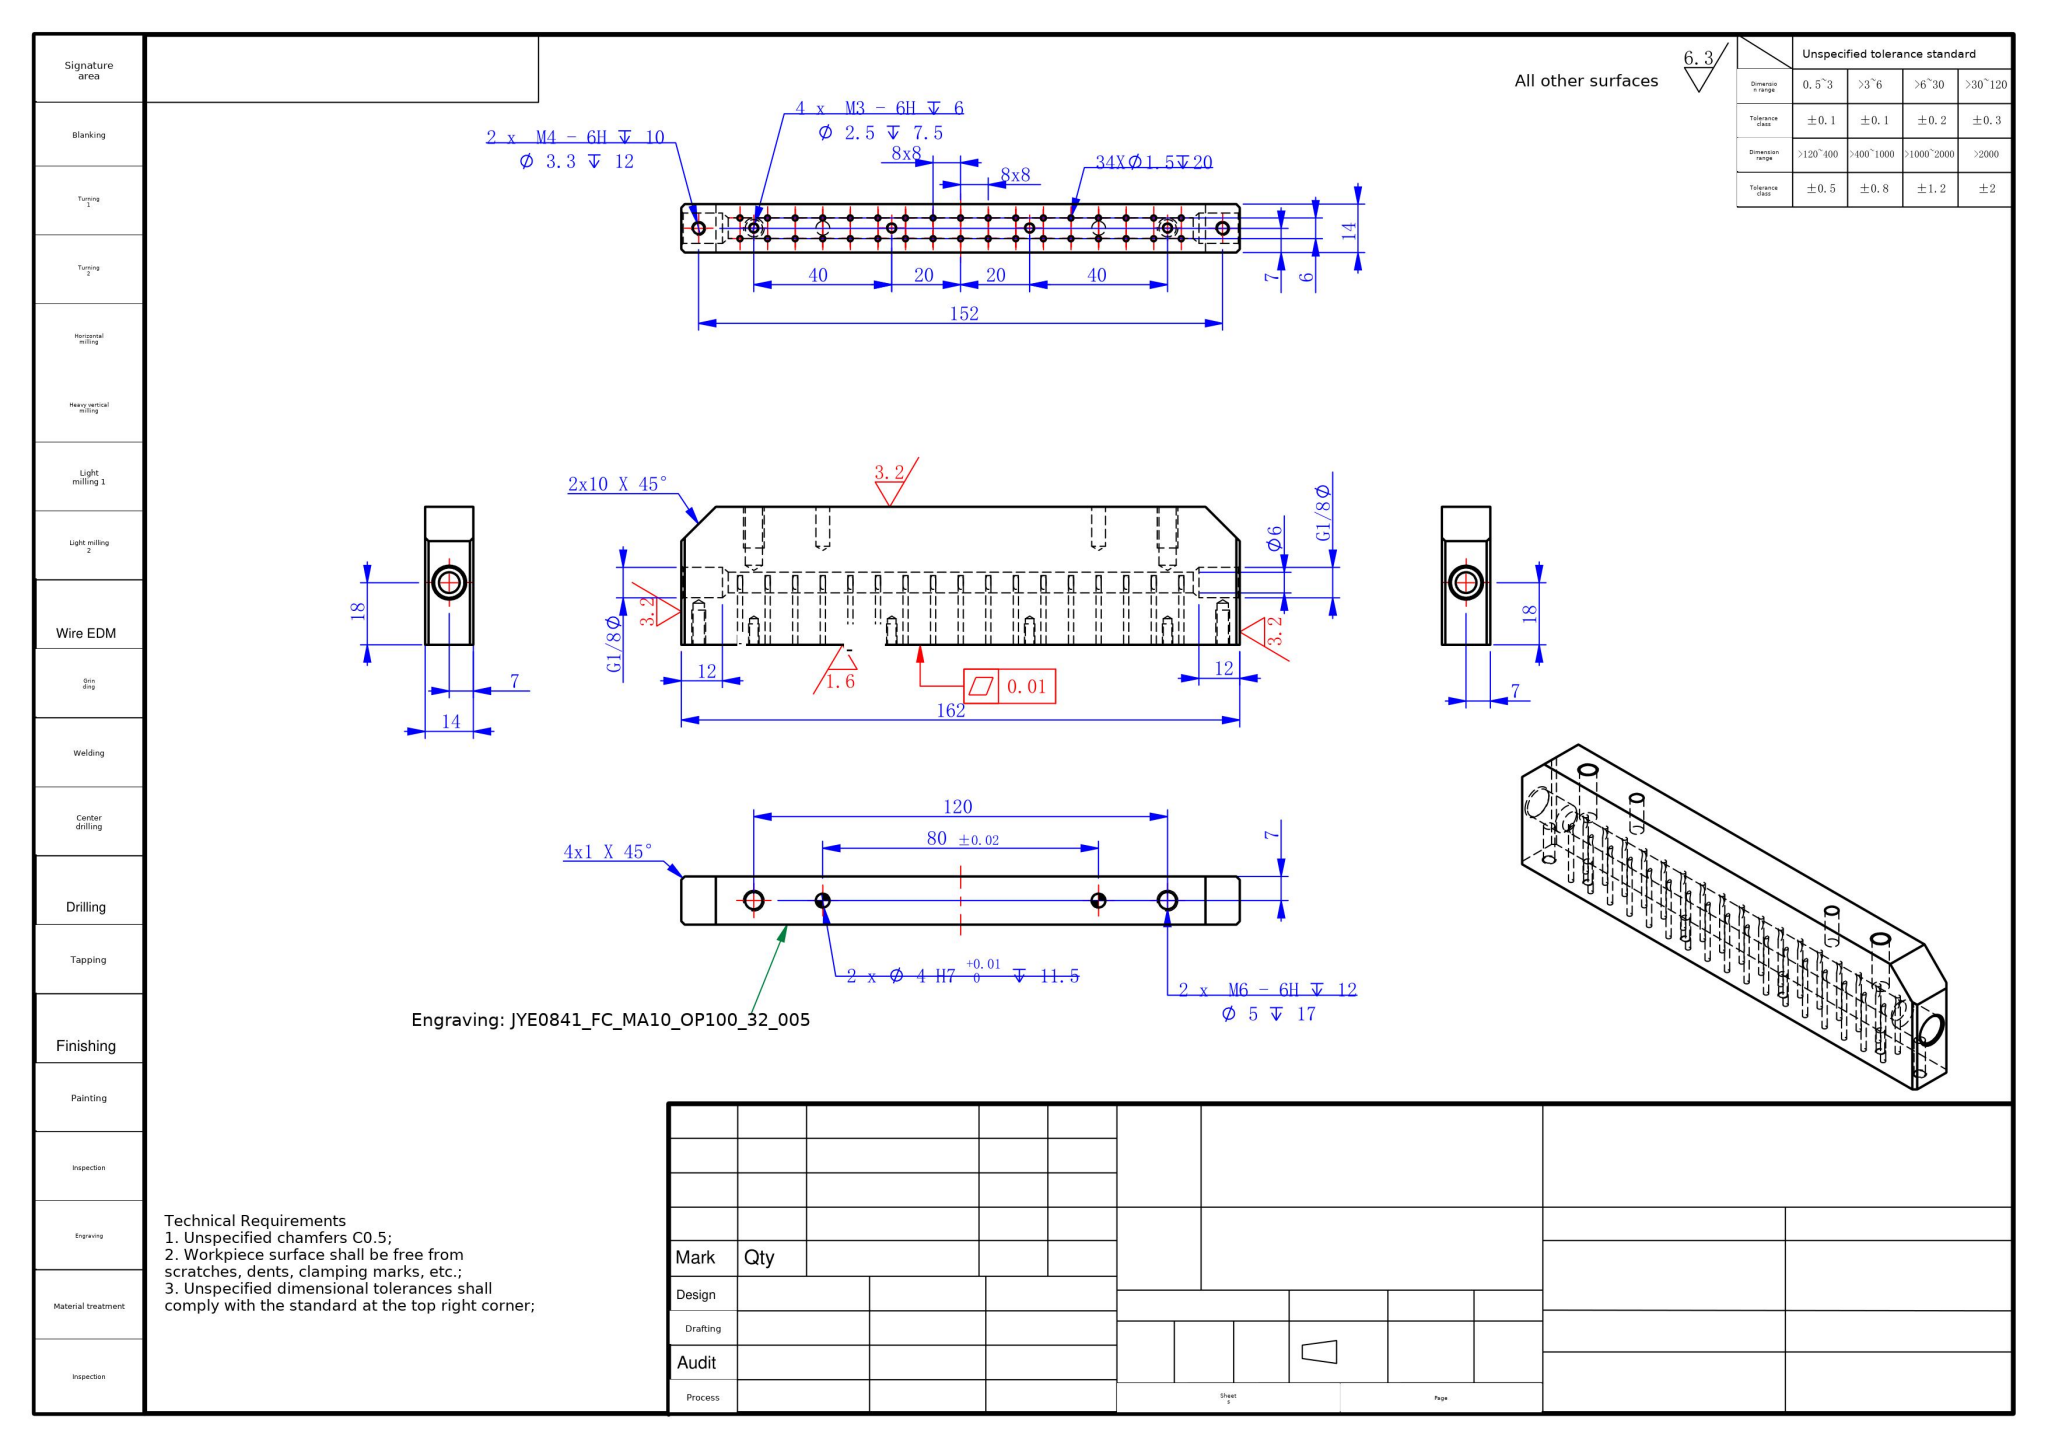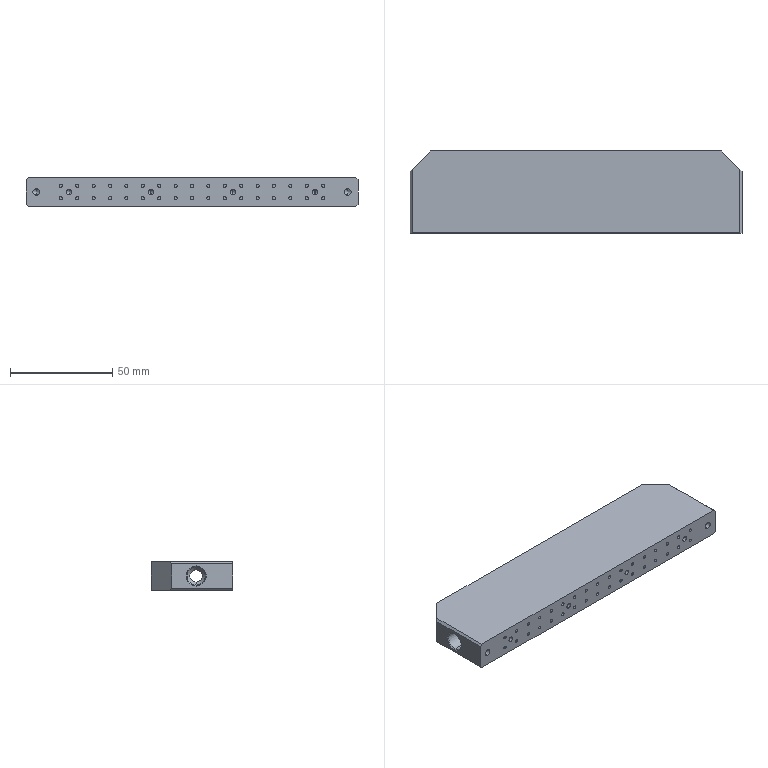Part | SolidWorks | mm | 1 solid | 168 faces | box 162 x 40 x 14 mm | volume 81371 mm3 | cylinder 94 | plane 46 | cone 28 | commonest cylinder face diameters 1.5 x68 2.5 x8 3.3 x4 5 x4 4 x4 8.8 x4 6 x2
build123d program:
from build123d import *

# Parameters (mm, degrees)
BOSS_EXTRUDE1_DEPTH          = 14
F_4_0_4_DIAMETER_HOLE1_D     = 4
F_4_0_4_DIAMETER_HOLE1_DEPTH = 11.5
F_4_0_4_DIAMETER_HOLE1_TIP   = 1.202
CHAMFER2_SIZE                = 0.489
CHAMFER3_SIZE                = 1
SKETCH11_R                   = 0.75
CUT_EXTRUDE1_DEPTH           = 20
LPATTERN1_COUNT              = 9
LPATTERN1_PITCH              = 8
LPATTERN1_COL_COUNT          = 9
LPATTERN1_COL_PITCH          = 8
M3_TAPPED_HOLE1_D            = 2.5
M3_TAPPED_HOLE1_DEPTH        = 7.5
M3_TAPPED_HOLE1_TIP          = 0.7511
M6_TAPPED_HOLE1_D            = 5
M6_TAPPED_HOLE1_DEPTH        = 17
M6_TAPPED_HOLE1_TIP          = 1.502
M4_TAPPED_HOLE1_D            = 3.3
M4_TAPPED_HOLE1_DEPTH        = 12
M4_TAPPED_HOLE1_TIP          = 0.9914


with BuildPart() as part:
    # Sketch1 → Boss-Extrude1 (new body)
    with BuildSketch(Plane.XY.offset(7)):
        Polygon((-71, 0), (-81, -10), (-81, -40), (81, -40), (81, -10), (71, 0), align=None)
    extrude(amount=-BOSS_EXTRUDE1_DEPTH)

    # Sketch2 → Cut-Revolve1 (revolve, cut)
    with BuildSketch(Plane(origin=(0, 0, 0), x_dir=(-1, 0, 0), z_dir=(0, 0, -1)), mode=Mode.PRIVATE) as cut_revolve1_sk:
        Polygon((-81, -17.6), (-81, -22), (81, -22), (81, -17.6), (69.108, -17.6), (67.44, -19), (-67.439, -19), (-69.107, -17.6), align=None)
    revolve(cut_revolve1_sk.sketch.rotate(Axis((81, -22, 0), (-1, 0, 0)), 270), axis=Axis((81, -22, 0), (-1, 0, 0)), mode=Mode.SUBTRACT)

    # 4.0 _4_ Diameter Hole1
    with Locations(Plane(origin=(0, 0, 0), x_dir=(1, 0, 0), z_dir=(0, 1, 0))):
        with Locations((40, 0), (-40, 0)):
            Hole(F_4_0_4_DIAMETER_HOLE1_D / 2, depth=F_4_0_4_DIAMETER_HOLE1_DEPTH)
            with Locations((0, 0, -(F_4_0_4_DIAMETER_HOLE1_DEPTH + F_4_0_4_DIAMETER_HOLE1_TIP / 2))):  # 118° drill point
                Cone(0, F_4_0_4_DIAMETER_HOLE1_D / 2, F_4_0_4_DIAMETER_HOLE1_TIP, mode=Mode.SUBTRACT)

    # Chamfer2
    chamfer2_edges = [part.edges().sort_by_distance(p)[0] for p in [
        (81, -22, -4.4),
        (-81, -22, -4.4),
    ]]
    chamfer(chamfer2_edges, length=CHAMFER2_SIZE)

    # Chamfer3
    chamfer3_edges = [part.edges().sort_by_distance(p)[0] for p in [
        (-81, -25, -7),
        (81, -25, -7),
        (81, -25, 7),
        (-81, -25, 7),
    ]]
    chamfer(chamfer3_edges, length=CHAMFER3_SIZE)

    # Sketch11 → Cut-Extrude1 (cut)
    with BuildSketch(Plane.XZ.offset(40)):
        with Locations(Location((0, 3, 0), (0, 0, 270))):
            Circle(SKETCH11_R)
        with Locations(Location((0, -3, 0), (0, 0, 270))):
            Circle(SKETCH11_R)
    cut_extrude1 = extrude(amount=-CUT_EXTRUDE1_DEPTH, mode=Mode.SUBTRACT)

    # LPattern1: Cut-Extrude1 ×9
    with Locations(*[(i * LPATTERN1_PITCH, 0, 0) for i in range(1, LPATTERN1_COUNT)]):
        add(cut_extrude1, mode=Mode.SUBTRACT)

    # LPattern1 col: Cut-Extrude1 ×9
    with Locations(*[(-i * LPATTERN1_COL_PITCH, 0, 0) for i in range(1, LPATTERN1_COL_COUNT)]):
        add(cut_extrude1, mode=Mode.SUBTRACT)

    # M3 Tapped Hole1
    with Locations(Plane(origin=(0, -40, 0), x_dir=(-1, 0, 0), z_dir=(0, -1, 0))):
        with Locations((-60, 0.08509), (-20, 0.08509), (20, 0.08509), (60, 0.08509)):
            Hole(M3_TAPPED_HOLE1_D / 2, depth=M3_TAPPED_HOLE1_DEPTH)
            with Locations((0, 0, -(M3_TAPPED_HOLE1_DEPTH + M3_TAPPED_HOLE1_TIP / 2))):  # 118° drill point
                Cone(0, M3_TAPPED_HOLE1_D / 2, M3_TAPPED_HOLE1_TIP, mode=Mode.SUBTRACT)

    # M6 Tapped Hole1
    with Locations(Plane(origin=(0, 0, 0), x_dir=(1, 0, 0), z_dir=(0, 1, 0))):
        with Locations((-60, 0), (60, 0)):
            Hole(M6_TAPPED_HOLE1_D / 2, depth=M6_TAPPED_HOLE1_DEPTH)
            with Locations((0, 0, -(M6_TAPPED_HOLE1_DEPTH + M6_TAPPED_HOLE1_TIP / 2))):  # 118° drill point
                Cone(0, M6_TAPPED_HOLE1_D / 2, M6_TAPPED_HOLE1_TIP, mode=Mode.SUBTRACT)

    # M4 Tapped Hole1
    with Locations(Plane(origin=(0, -40, 0), x_dir=(-1, 0, 0), z_dir=(0, -1, 0))):
        with Locations((-76, 0), (76, 0)):
            Hole(M4_TAPPED_HOLE1_D / 2, depth=M4_TAPPED_HOLE1_DEPTH)
            with Locations((0, 0, -(M4_TAPPED_HOLE1_DEPTH + M4_TAPPED_HOLE1_TIP / 2))):  # 118° drill point
                Cone(0, M4_TAPPED_HOLE1_D / 2, M4_TAPPED_HOLE1_TIP, mode=Mode.SUBTRACT)


solid = part.part